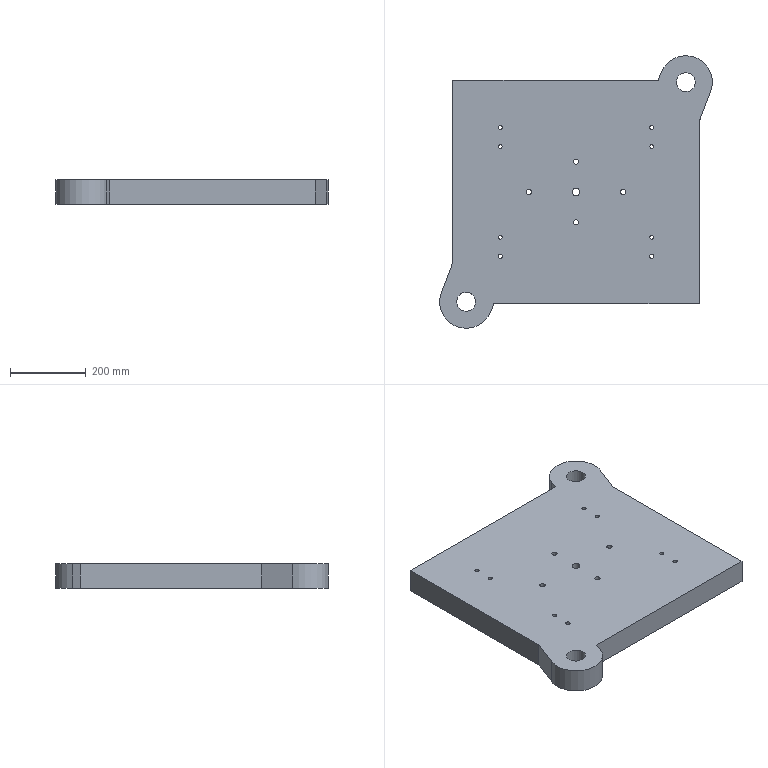Component | NX | LOWER_DIE_BASE | 1 solid | 38 faces | volume 25723786 mm3 | cylinder 22 | plane 15 | cone 1 | commonest cylinder face diameters 11 x4 18 x4 10 x4 14 x4 140 x2 50 x2 21 x1 32 x1